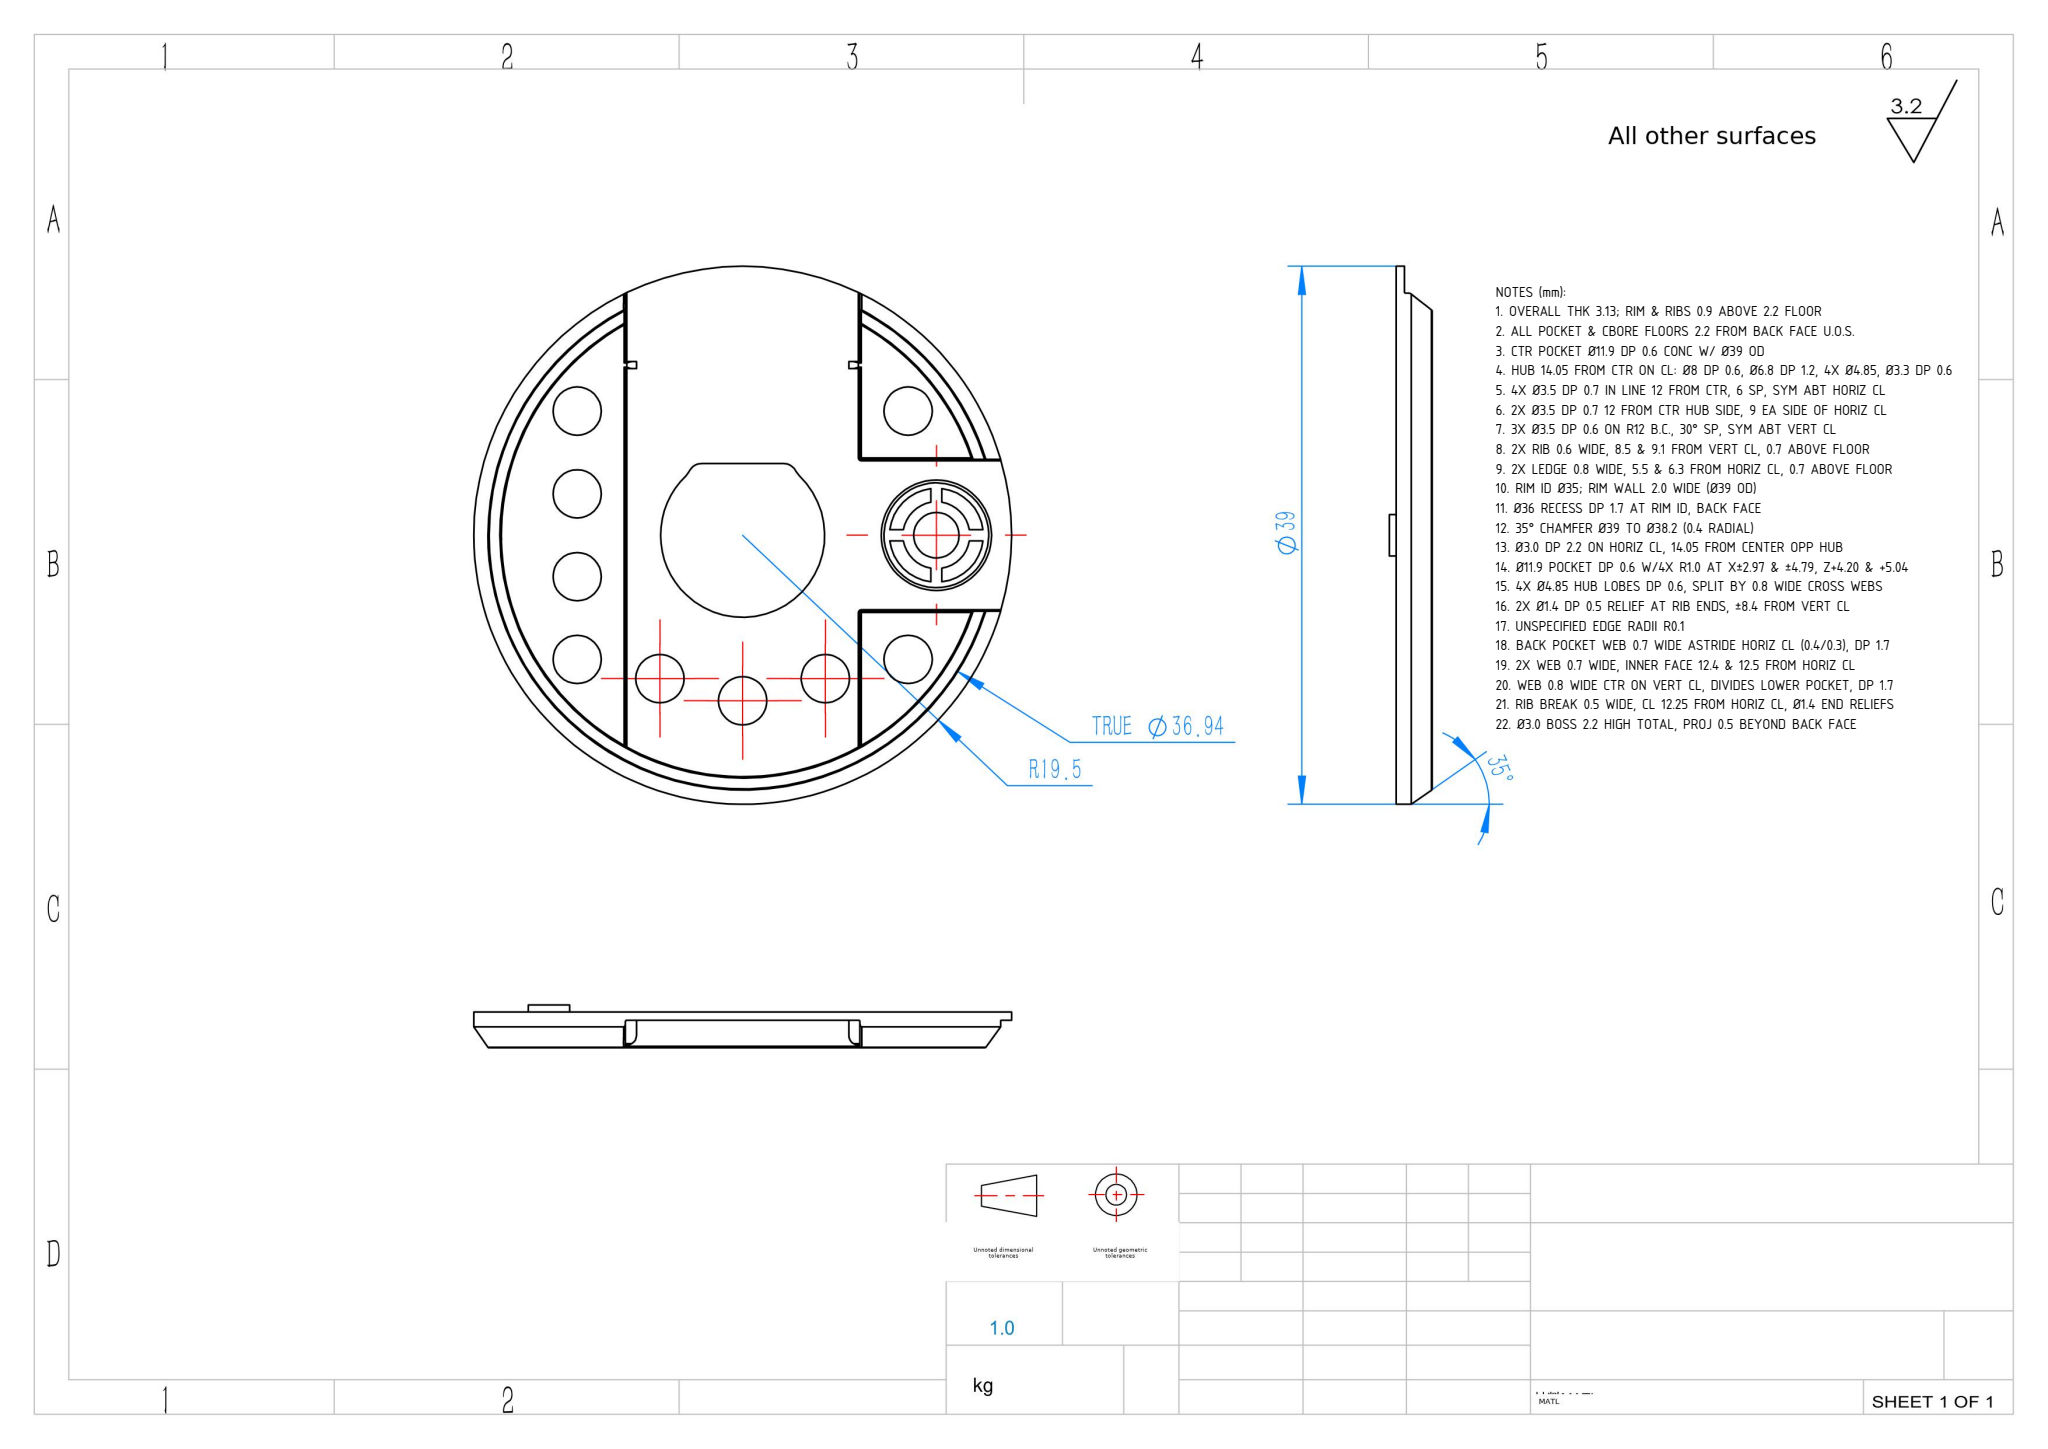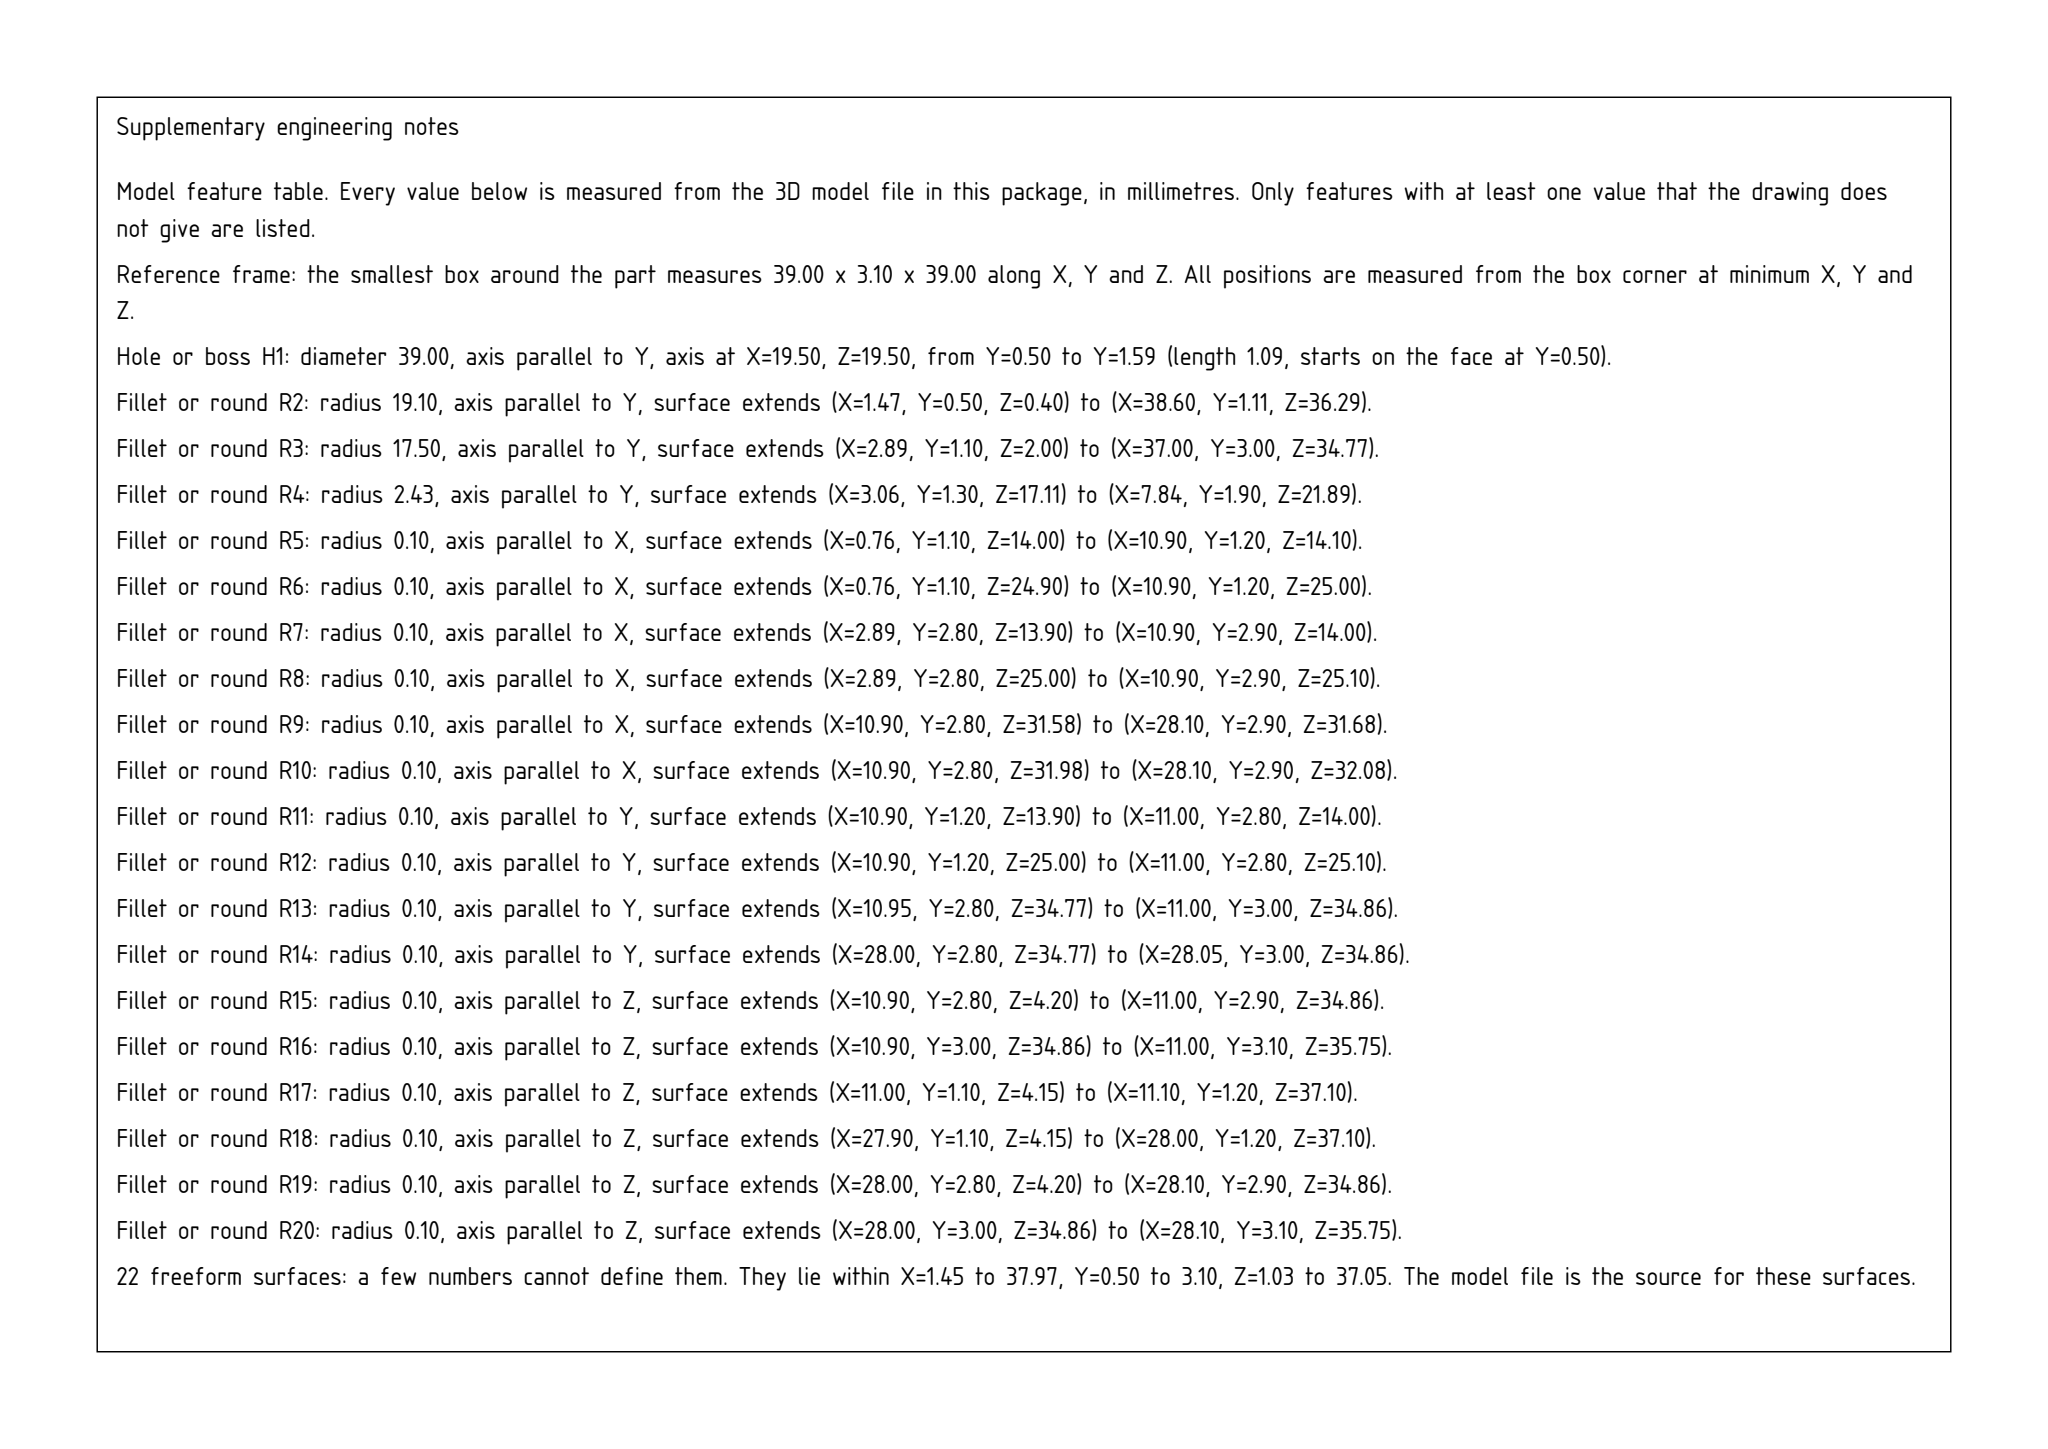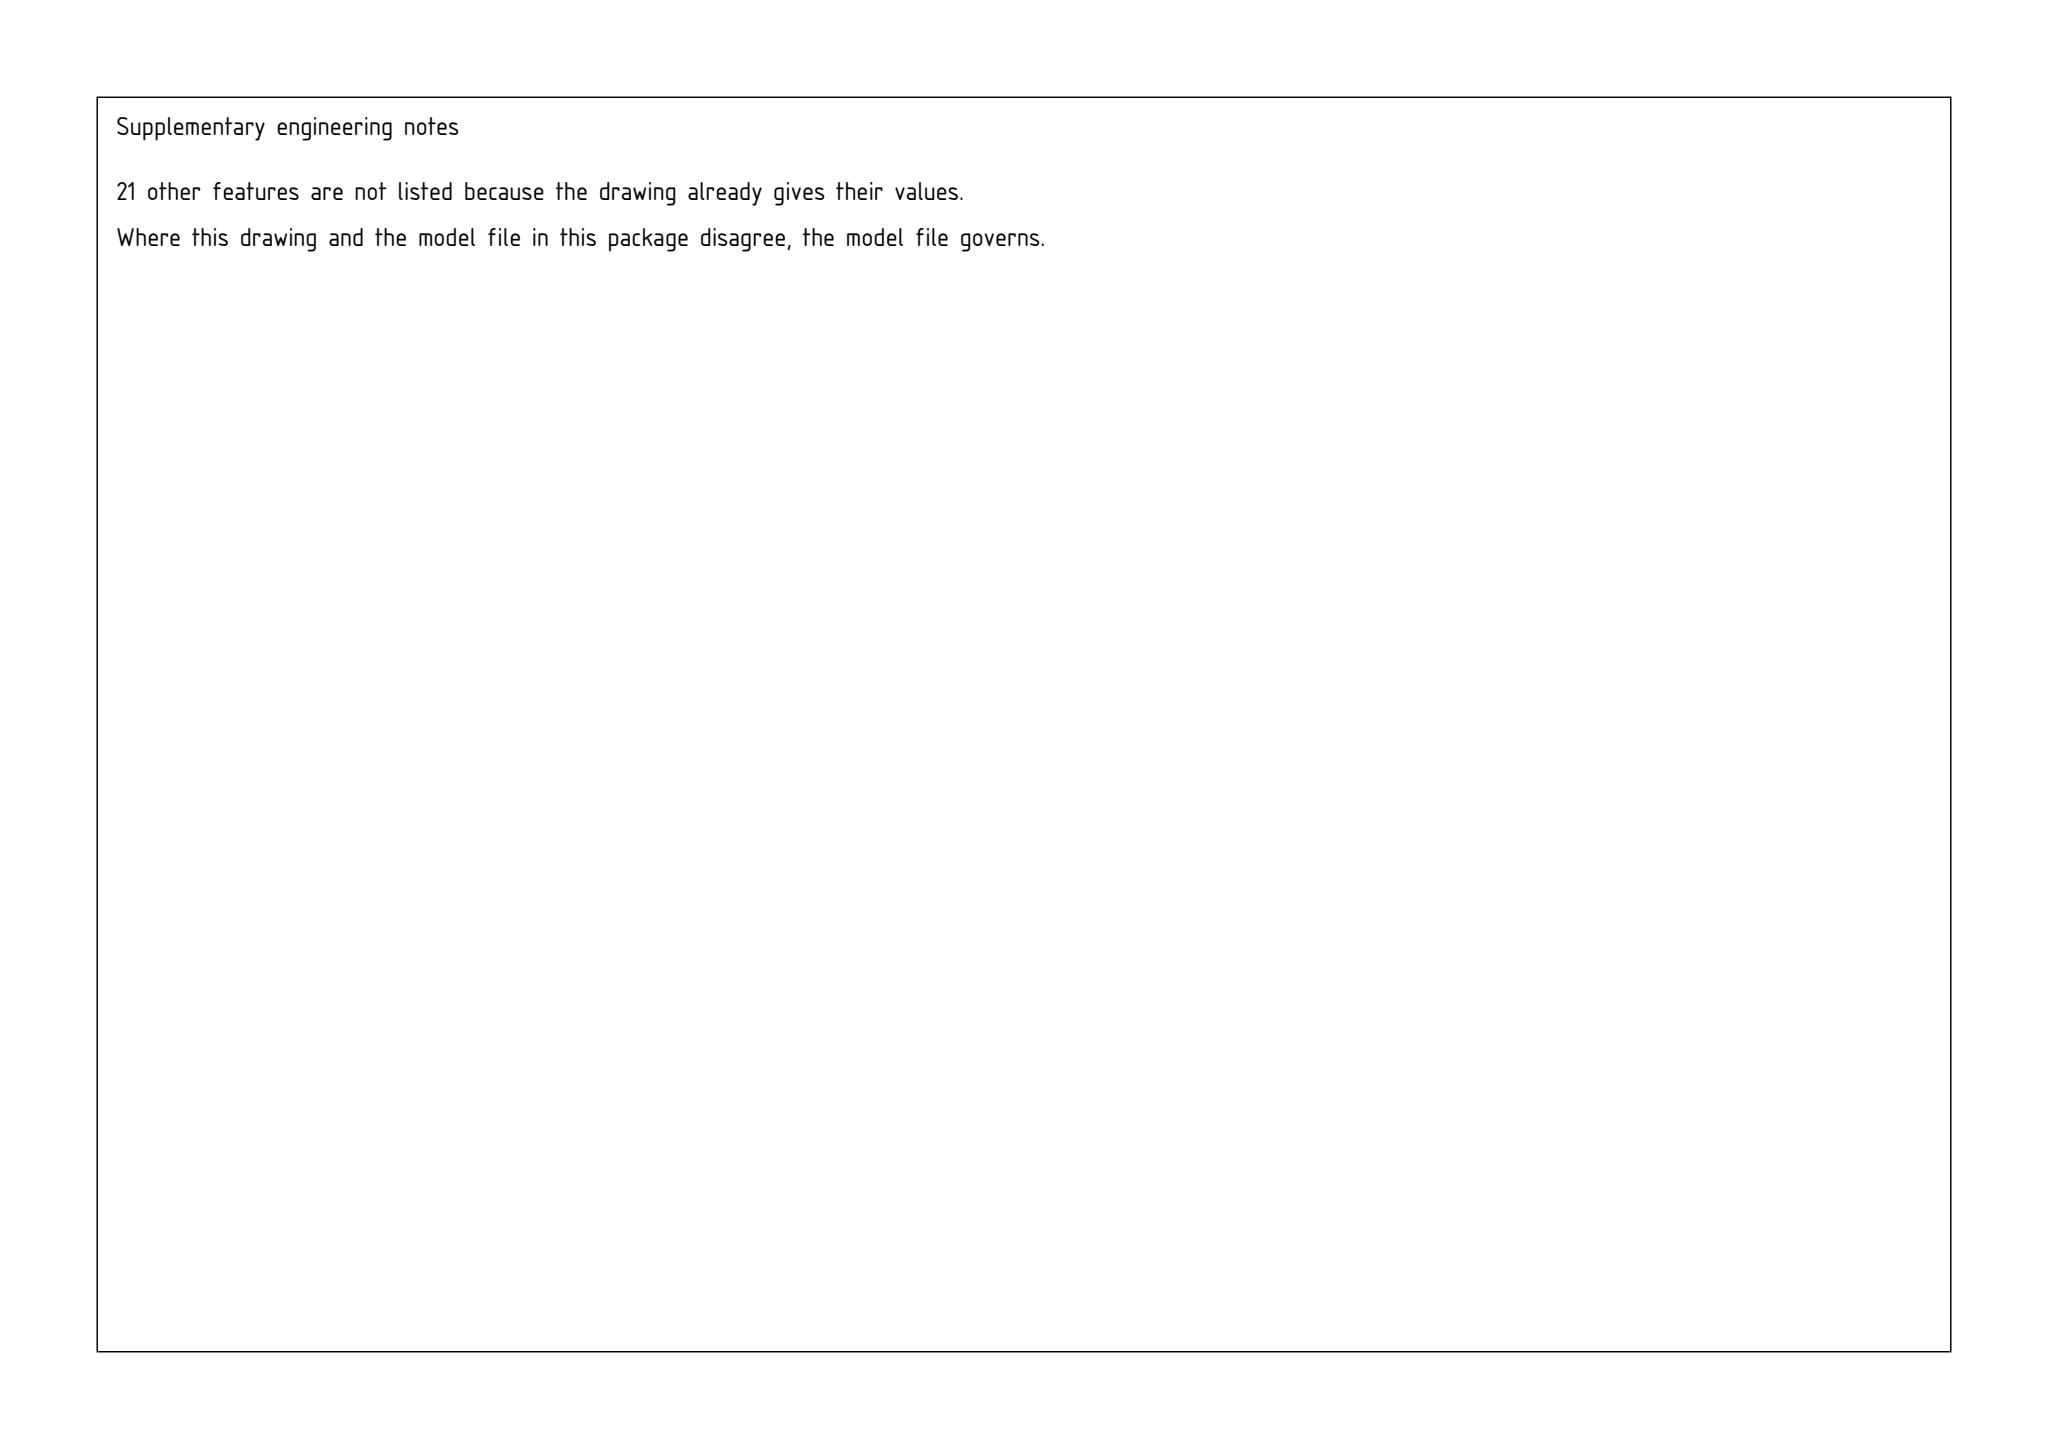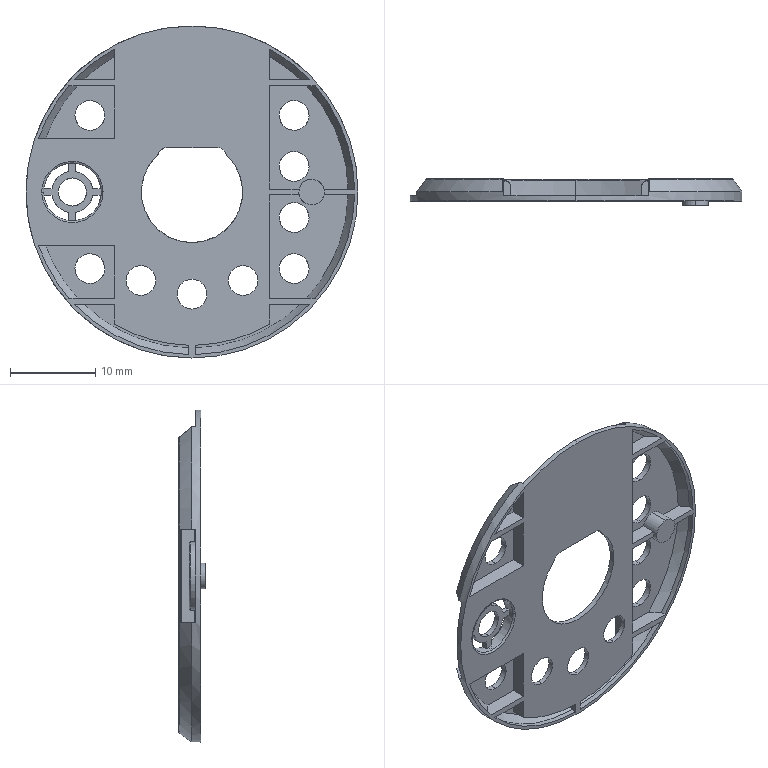Part | SolidWorks | mm | 1 solid | 173 faces | box 39 x 3.1 x 39 mm | volume 841 mm3 | cylinder 76 | plane 64 | spline 22 | cone 11 | commonest cylinder face diameters 0.2 x24 3.5 x18 38.2 x8 2 x4 4.85 x4 35 x3 39 x2 6.8 x2
Drawing notes:
OVERALL THK 3.13; RIM & RIBS 0.9 ABOVE 2.2 FLOOR | from the solid: bbox y=3.133; y-planes 0.0/2.2/3.1 -> floor 2.2, top 3.1 (0.9 high)
ALL POCKET & CBORE FLOORS 2.2 FROM BACK FACE U.O.S. | from the solid: y-plane 2.2 occurs 8X (main recessed floor); pocket depths 0.6/0.7 to it
CTR POCKET Ø11.9 DP 0.6 CONC W/ Ø39 OD | from the solid: Ø11.9 y-cyl at (19.5,23.65) len 0.6, coaxial with Ø39 disc
HUB 14.05 FROM CTR ON CL: Ø8 DP 0.6, Ø6.8 DP 1.2, 4X Ø4.85, Ø3.3 DP 0.6 | from the solid: coaxial y-cyls at (5.45,23.65): Ø8 L0.6, Ø6.8 L1.2, 4X Ø4.85 L0.6, Ø3.3 L0.6; 19.5-5.45=14.05
4X Ø3.5 DP 0.7 IN LINE 12 FROM CTR, 6 SP, SYM ABT HORIZ CL | from the solid: Ø3.5 y-cyls x=31.5, z=14.65/20.65/26.65/32.65, L0.7; ctr (19.5,23.65)
2X Ø3.5 DP 0.7 12 FROM CTR HUB SIDE, 9 EA SIDE OF HORIZ CL | from the solid: Ø3.5 y-cyls at (7.5,14.65) & (7.5,32.65), L0.7; 12 from ctr x, 9 from ctr z
3X Ø3.5 DP 0.6 ON R12 B.C., 30° SP, SYM ABT VERT CL | from the solid: Ø3.5 y-cyls (13.5,13.26),(19.5,11.65),(25.5,13.26) L0.6; R12 from ctr, 30° apart
2X RIB 0.6 WIDE, 8.5 & 9.1 FROM VERT CL, 0.7 ABOVE FLOOR | from the solid: x-planes 10.4/11.0 and 28.0/28.6 (ctr x=19.5); y 2.2 to 2.9
2X LEDGE 0.8 WIDE, 5.5 & 6.3 FROM HORIZ CL, 0.7 ABOVE FLOOR | from the solid: z-planes 17.35/18.15 and 29.15/29.95 (ctr z=23.65); y 2.2 to 2.9
RIM ID Ø35; RIM WALL 2.0 WIDE (Ø39 OD) | from the solid: cyl Ø35 y-axis @ (19.5,23.65) vs Ø39 OD: (39-35)/2=2.0
Ø36 RECESS DP 1.7 AT RIM ID, BACK FACE | from the solid: cyl [36.0,'y',[19.5,23.65],1.7] step between Ø39 and Ø35
35° CHAMFER Ø39 TO Ø38.2 (0.4 RADIAL) | from the solid: cones [70.0,39.0] & [70.0,38.2]; half angle 35°, (39-38.2)/2=0.4
Ø3.0 DP 2.2 ON HORIZ CL, 14.05 FROM CENTER OPP HUB | from the solid: cyl [3.0,'y',[33.55,23.65],2.2]; 33.55-19.5=14.05, same Z as CL
Ø11.9 POCKET DP 0.6 W/4X R1.0 AT X±2.97 & ±4.79, Z+4.20 & +5.04 | from the solid: cyl Ø11.9 x0.6 @ (19.5,23.65); 4X Ø2.0 x0.6 @ (16.53/22.47,27.85) & (14.71/24.29,28.69)
4X Ø4.85 HUB LOBES DP 0.6, SPLIT BY 0.8 WIDE CROSS WEBS | from the solid: 4X cyl Ø4.85 @ (5.45,23.65) L0.6; planes x=5.05/5.85 & z=23.25/24.05 = ±0.4 from hub CL
2X Ø1.4 DP 0.5 RELIEF AT RIB ENDS, ±8.4 FROM VERT CL | from the solid: cyl [1.4,'z',[11.1,2.2],0.5] & [1.4,'z',[27.9,2.2],0.5]; 19.5-11.1=8.4
UNSPECIFIED EDGE RADII R0.1 | from the solid: all 0.2 dia fillet cylinders on rib/ledge/pocket edges = R0.1
BACK POCKET WEB 0.7 WIDE ASTRIDE HORIZ CL (0.4/0.3), DP 1.7 | from the solid: Planes z=23.3 & z=24.0, x[28.6,32.1] & x[35.0,38.6], y[0.5,2.2]; part CL z=23.7; pocket flr y=2.2 vs back face y=0.5
2X WEB 0.7 WIDE, INNER FACE 12.4 & 12.5 FROM HORIZ CL | from the solid: Planes z=10.5/11.2 and z=36.1/36.8 bounding y=2.2 pocket floors; CL z=23.7 -> 23.7-11.2=12.5, 36.1-23.7=12.4
WEB 0.8 WIDE CTR ON VERT CL, DIVIDES LOWER POCKET, DP 1.7 | from the solid: Planes x=19.1 & x=19.9, y[0.5,2.2]; vert CL x=19.5; floors y=2.2 x[6.8,19.1] & x[19.9,32.2], z[5.3,10.5]
RIB BREAK 0.5 WIDE, CL 12.25 FROM HORIZ CL, Ø1.4 END RELIEFS | from the solid: Ø1.4 convex arcs, axis z at x=11.1 & 27.9, z 35.7-36.2; mid z=35.95; horiz CL z=23.7
Ø3.0 BOSS 2.2 HIGH TOTAL, PROJ 0.5 BEYOND BACK FACE | from the solid: Ø3.0 cyl axis y at (33.6,23.7), y 0.0-2.2; back face plane y=0.5; top face y=0.0 x[32.1,35.1] z[22.2,25.2]